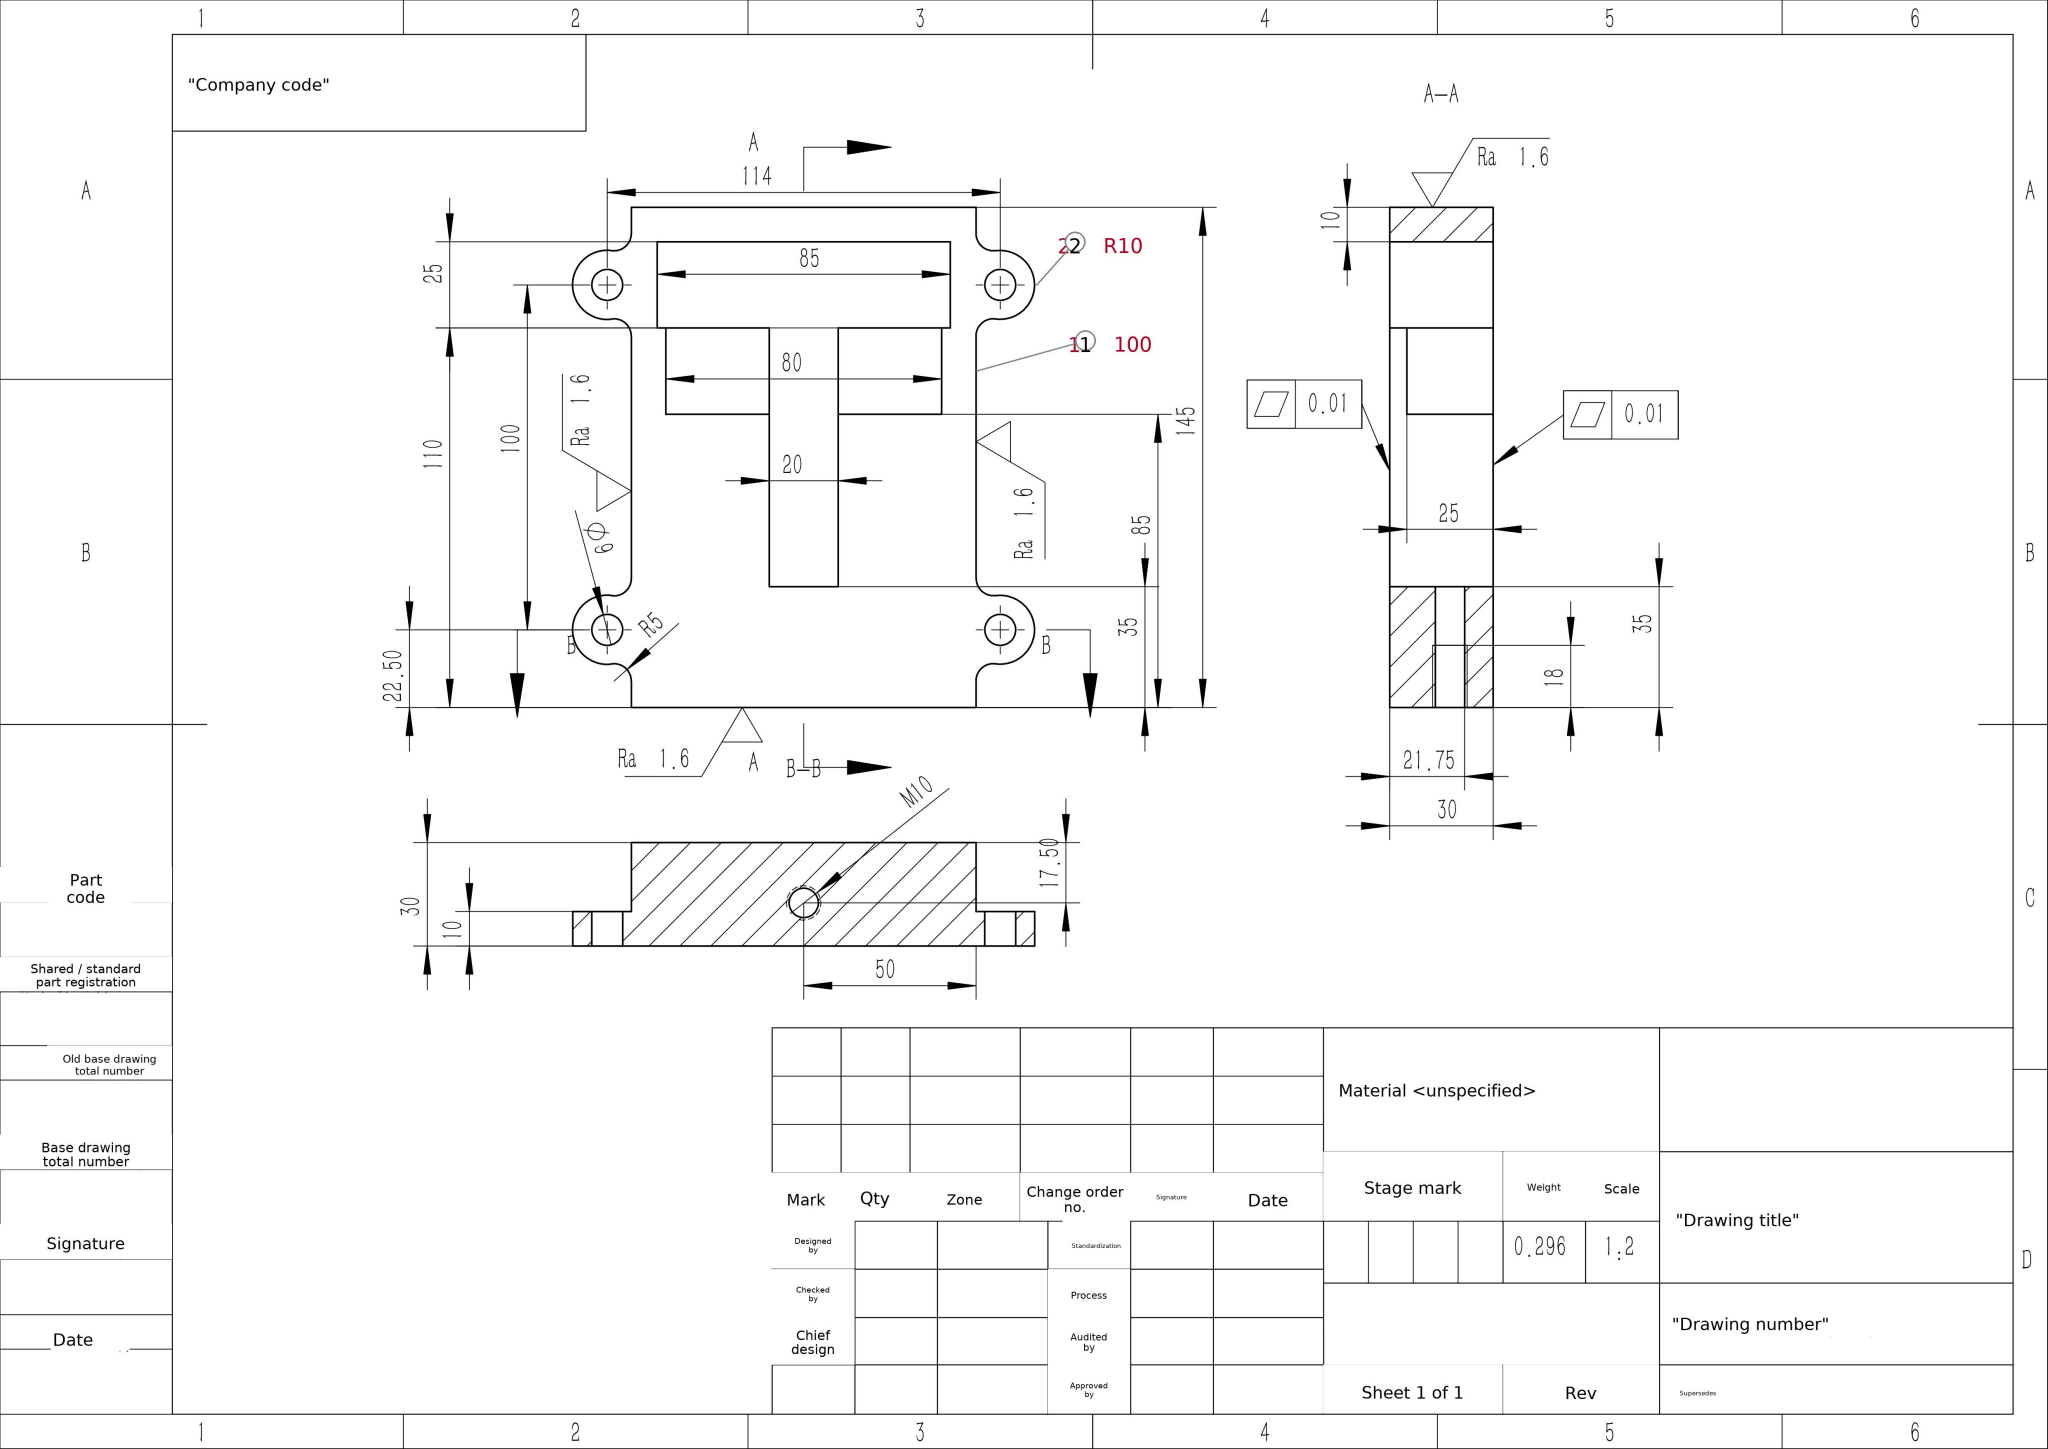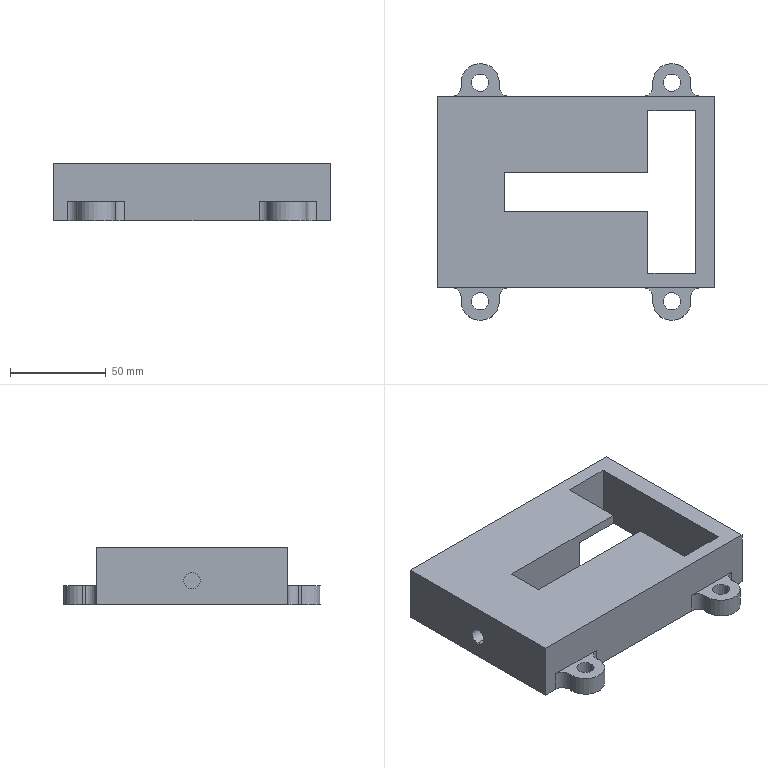Part | SolidWorks | mm | 1 solid | 58 faces | box 145 x 134 x 30 mm | volume 296469 mm3 | cylinder 34 | plane 24 | commonest cylinder face diameters 10 x12 20 x12 9 x8 8.5 x2
build123d program:
from build123d import *

# Parameters (mm, degrees)
SKETCH1_W              = 35
SKETCH1_H              = 90
SKETCH1_W_2            = 25
SKETCH1_H_2            = 80
BOSS_EXTRUDE1_DEPTH    = 30
SKETCH2_W              = 100
SKETCH2_H              = 90
BOSS_EXTRUDE2_DEPTH    = 30
SKETCH3_W              = 145
SKETCH3_H              = 100
SKETCH3_W_2            = 25
SKETCH3_H_2            = 80
BOSS_EXTRUDE3_DEPTH    = 30
SKETCH4_R              = 10
BOSS_EXTRUDE4_DEPTH    = 10
FILLET1_R              = 5
SKETCH5_R              = 4.5
CUT_EXTRUDE1_DEPTH     = 10
SKETCH6_W              = 100
SKETCH6_H              = 20
CUT_EXTRUDE2_DEPTH     = 143.812
SKETCH7_W              = 25
SKETCH7_H              = 80
CUT_EXTRUDE3_DEPTH     = 25
SKETCH8_W              = 25
SKETCH8_H              = 20
BOSS_EXTRUDE5_DEPTH    = 30
M10_TAPPED_HOLE1_D     = 8.5
M10_TAPPED_HOLE1_DEPTH = 52.5
M10_TAPPED_HOLE1_TIP   = 2.554
SKETCH13_W             = 25
SKETCH13_H             = 85
CUT_EXTRUDE4_DEPTH     = 143.812


with BuildPart() as part:
    # Sketch1 → Boss-Extrude1 (new body)
    with BuildSketch(Plane.XY):
        Rectangle(SKETCH1_W, SKETCH1_H)
        Rectangle(SKETCH1_W_2, SKETCH1_H_2, mode=Mode.SUBTRACT)
    extrude(amount=BOSS_EXTRUDE1_DEPTH)

    # Sketch2 → Boss-Extrude2 (add)
    with BuildSketch(Plane.XY.offset(30)):
        with Locations((-67.5, 0)):
            Rectangle(SKETCH2_W, SKETCH2_H)
    extrude(amount=-BOSS_EXTRUDE2_DEPTH)

    # Sketch3 → Boss-Extrude3 (add)
    with BuildSketch(Plane.XY.offset(30)):
        with Locations((-50, 0)):
            Rectangle(SKETCH3_W, SKETCH3_H)
        Rectangle(SKETCH3_W_2, SKETCH3_H_2, mode=Mode.SUBTRACT)
    extrude(amount=-BOSS_EXTRUDE3_DEPTH)

    # Sketch4 → Boss-Extrude4 (add)
    with BuildSketch(Plane(origin=(0, 0, 0), x_dir=(-1, 0, 0), z_dir=(0, 0, -1))):
        with Locations((100, 57)):
            Circle(SKETCH4_R)
        with Locations((100, -57)):
            Circle(SKETCH4_R)
        with Locations((0, -57)):
            Circle(SKETCH4_R)
        with Locations((0, 57)):
            Circle(SKETCH4_R)
    extrude(amount=-BOSS_EXTRUDE4_DEPTH)

    # Fillet1
    fillet1_edges = [part.edges().sort_by_distance(p)[0] for p in [
        (-107.141, 50, 5),
        (-92.859, 50, 5),
        (-92.859, -50, 5),
        (-107.141, -50, 5),
        (7.141, -50, 5),
        (-7.141, -50, 5),
        (-7.141, 50, 5),
        (7.141, 50, 5),
    ]]
    fillet(fillet1_edges, radius=FILLET1_R)

    # Sketch5 → Cut-Extrude1 (cut)
    with BuildSketch(Plane.XY.offset(10)):
        with Locations((-100, 57)):
            Circle(SKETCH5_R)
        with Locations((-100, -57)):
            Circle(SKETCH5_R)
        with Locations(Location((0, -57, 0), (0, 0, 180))):
            Circle(SKETCH5_R)
        with Locations(Location((0, 57, 0), (0, 0, 180))):
            Circle(SKETCH5_R)
    extrude(amount=-CUT_EXTRUDE1_DEPTH, mode=Mode.SUBTRACT)

    # Sketch6 → Cut-Extrude2 (cut, through all)
    with BuildSketch(Plane.XY.offset(30)):
        with Locations((-62.5, 0)):
            Rectangle(SKETCH6_W, SKETCH6_H)
    extrude(amount=-CUT_EXTRUDE2_DEPTH, mode=Mode.SUBTRACT)

    # Sketch7 → Cut-Extrude3 (cut)
    with BuildSketch(Plane(origin=(0, 0, 0), x_dir=(-1, 0, 0), z_dir=(0, 0, -1))):
        with Locations((25, 0)):
            Rectangle(SKETCH7_W, SKETCH7_H)
    extrude(amount=-CUT_EXTRUDE3_DEPTH, mode=Mode.SUBTRACT)

    # Sketch8 → Boss-Extrude5 (add)
    with BuildSketch(Plane(origin=(0, 0, 0), x_dir=(-1, 0, 0), z_dir=(0, 0, -1))):
        with Locations((100, 0)):
            Rectangle(SKETCH8_W, SKETCH8_H)
    extrude(amount=-BOSS_EXTRUDE5_DEPTH)

    # M10 Tapped Hole1
    with Locations(Plane.ZY.offset(122.5)):
        with Locations((12.5, 0)):
            Hole(M10_TAPPED_HOLE1_D / 2, depth=M10_TAPPED_HOLE1_DEPTH)
            with Locations((0, 0, -(M10_TAPPED_HOLE1_DEPTH + M10_TAPPED_HOLE1_TIP / 2))):  # 118° drill point
                Cone(0, M10_TAPPED_HOLE1_D / 2, M10_TAPPED_HOLE1_TIP, mode=Mode.SUBTRACT)

    # Sketch13 → Cut-Extrude4 (cut, through all)
    with BuildSketch(Plane.XY.offset(30)):
        Rectangle(SKETCH13_W, SKETCH13_H)
    extrude(amount=-CUT_EXTRUDE4_DEPTH, mode=Mode.SUBTRACT)


solid = part.part